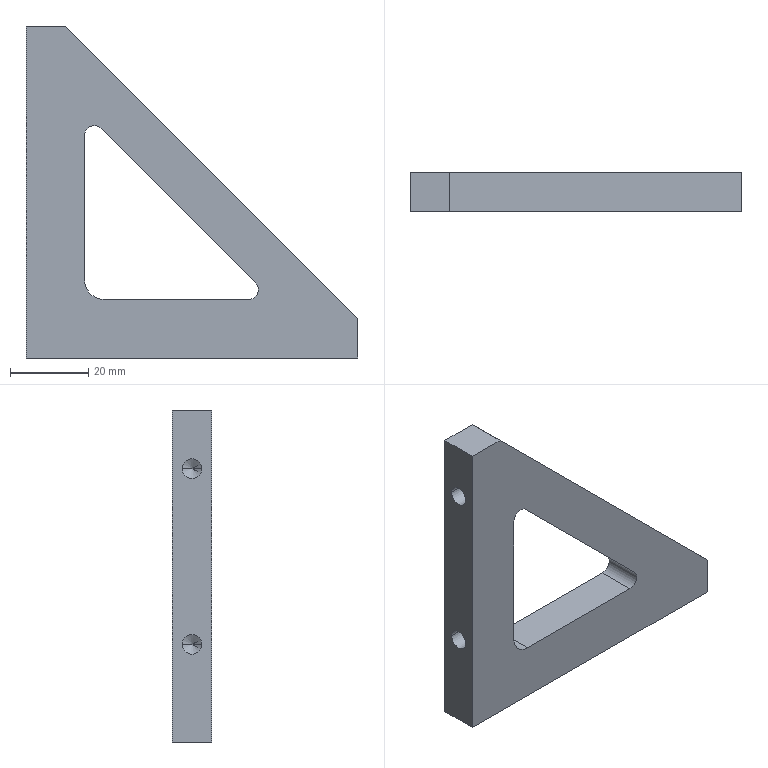Component | SolidWorks | 17081801-804-015A-1 | 1 solid | 29 faces | box 85 x 10 x 85 mm | volume 31739 mm3 | cylinder 11 | plane 10 | cone 8 | commonest cylinder face diameters 5 x10 10 x1 | material AL6061
build123d program:
from build123d import *

# Parameters (mm, degrees)
BOSS_EXTRUDE1_DEPTH   = 5
M6_TAPPED_HOLE2_D     = 5
M6_TAPPED_HOLE2_DEPTH = 13
M6_TAPPED_HOLE2_TIP   = 1.502
M6_TAPPED_HOLE1_D     = 5
M6_TAPPED_HOLE1_DEPTH = 13
M6_TAPPED_HOLE1_TIP   = 1.502
CUT_EXTRUDE1_DEPTH    = 121.623


with BuildPart() as part:
    # Sketch1 → Boss-Extrude1 (new, symmetric)
    with BuildSketch(Plane.XY):
        Polygon((0, 0), (85, 0), (85, 10), (10, 85), (0, 85), align=None)
    extrude(amount=BOSS_EXTRUDE1_DEPTH, both=True)

    # M6 Tapped Hole2
    with Locations(Plane(origin=(0, 0, 0), x_dir=(-1, 0, 0), z_dir=(0, -1, 0))):
        with Locations((-72, 0), (-27, 0)):
            Hole(M6_TAPPED_HOLE2_D / 2, depth=M6_TAPPED_HOLE2_DEPTH)
            with Locations((0, 0, -(M6_TAPPED_HOLE2_DEPTH + M6_TAPPED_HOLE2_TIP / 2))):  # 118° drill point
                Cone(0, M6_TAPPED_HOLE2_D / 2, M6_TAPPED_HOLE2_TIP, mode=Mode.SUBTRACT)

    # M6 Tapped Hole1
    with Locations(Plane(origin=(0, 0, 0), x_dir=(0, 0, -1), z_dir=(-1, 0, 0))):
        with Locations((0, -25), (0, -70)):
            Hole(M6_TAPPED_HOLE1_D / 2, depth=M6_TAPPED_HOLE1_DEPTH)
            with Locations((0, 0, -(M6_TAPPED_HOLE1_DEPTH + M6_TAPPED_HOLE1_TIP / 2))):  # 118° drill point
                Cone(0, M6_TAPPED_HOLE1_D / 2, M6_TAPPED_HOLE1_TIP, mode=Mode.SUBTRACT)

    # Sketch6 → Cut-Extrude1 (cut, through all)
    with BuildSketch(Plane(origin=(0, 0, -5), x_dir=(-1, 0, 0), z_dir=(0, 0, -1))):
        with BuildLine():
            Line((-58.762, 19.268), (-19.268, 58.762))
            ThreePointArc((-19.268, 58.762), (-16.543, 59.304), (-15, 56.994))
            Line((-15, 56.994), (-15, 20))
            ThreePointArc((-15, 20), (-16.464, 16.464), (-20, 15))
            Line((-20, 15), (-56.994, 15))
            ThreePointArc((-56.994, 15), (-59.304, 16.543), (-58.762, 19.268))
        make_face()
    extrude(amount=-CUT_EXTRUDE1_DEPTH, mode=Mode.SUBTRACT)


solid = part.part

# Placed as in the assembly
solid = solid.moved(Location((-116.5, 1974.4, 232), (90, 0, 0)))
STEP:
#1=COLOUR_RGB('',0.7922,0.8196,0.9333);
#2=FILL_AREA_STYLE_COLOUR('',#1);
#3=FILL_AREA_STYLE('',(#2));
#4=SURFACE_STYLE_FILL_AREA(#3);
#5=SURFACE_SIDE_STYLE('',(#4));
#6=SURFACE_STYLE_USAGE(.BOTH.,#5);
#7=PRESENTATION_STYLE_ASSIGNMENT((#6));
#8=CARTESIAN_POINT('',(-4.075,77.831,10.118));
#9=VERTEX_POINT('',#8);
#10=CARTESIAN_POINT('',(-4.075,77.634,10.118));
#11=VERTEX_POINT('',#10);
#12=CARTESIAN_POINT('',(-4.075,77.732,10.118));
#13=DIRECTION('',(-1.,0.,0.));
#14=DIRECTION('',(0.,-1.,0.));
#15=AXIS2_PLACEMENT_3D('',#12,#13,#14);
#16=CIRCLE('',#15,0.09843);
#17=EDGE_CURVE('',#9,#11,#16,.T.);
#18=ORIENTED_EDGE('',*,*,#17,.F.);
#19=CARTESIAN_POINT('',(-4.587,77.831,10.118));
#20=VERTEX_POINT('',#19);
#21=CARTESIAN_POINT('',(-4.587,77.831,10.118));
#22=DIRECTION('',(-1.,0.,0.));
#23=VECTOR('',#22,39.37);
#24=LINE('',#21,#23);
#25=EDGE_CURVE('',#9,#20,#24,.T.);
#26=ORIENTED_EDGE('',*,*,#25,.T.);
#27=CARTESIAN_POINT('',(-4.587,77.634,10.118));
#28=VERTEX_POINT('',#27);
#29=CARTESIAN_POINT('',(-4.587,77.732,10.118));
#30=DIRECTION('',(-1.,0.,0.));
#31=DIRECTION('',(0.,-1.,0.));
#32=AXIS2_PLACEMENT_3D('',#29,#30,#31);
#33=CIRCLE('',#32,0.09843);
#34=EDGE_CURVE('',#20,#28,#33,.T.);
#35=ORIENTED_EDGE('',*,*,#34,.T.);
#36=CARTESIAN_POINT('',(-4.587,77.634,10.118));
#37=DIRECTION('',(-1.,0.,0.));
#38=VECTOR('',#37,39.37);
#39=LINE('',#36,#38);
#40=EDGE_CURVE('',#11,#28,#39,.T.);
#41=ORIENTED_EDGE('',*,*,#40,.F.);
#42=EDGE_LOOP('',(#18,#26,#35,#41));
#43=FACE_OUTER_BOUND('',#42,.T.);
#44=CARTESIAN_POINT('',(-4.587,77.732,10.118));
#45=DIRECTION('',(-1.,0.,0.));
#46=DIRECTION('',(0.,-1.,0.));
#47=AXIS2_PLACEMENT_3D('',#44,#45,#46);
#48=CYLINDRICAL_SURFACE('',#47,0.09843);
#49=ADVANCED_FACE('',(#43),#48,.F.);
#50=CARTESIAN_POINT('',(-4.016,77.732,10.118));
#51=VERTEX_POINT('',#50);
#52=CARTESIAN_POINT('',(-4.075,77.634,10.118));
#53=DIRECTION('',(-0.515,-0.8572,-0.));
#54=VECTOR('',#53,39.37);
#55=LINE('',#52,#54);
#56=EDGE_CURVE('',#51,#11,#55,.T.);
#57=ORIENTED_EDGE('',*,*,#56,.F.);
#58=CARTESIAN_POINT('',(-4.075,77.831,10.118));
#59=DIRECTION('',(-0.515,0.8572,0.));
#60=VECTOR('',#59,39.37);
#61=LINE('',#58,#60);
#62=EDGE_CURVE('',#51,#9,#61,.T.);
#63=ORIENTED_EDGE('',*,*,#62,.T.);
#64=ORIENTED_EDGE('',*,*,#17,.T.);
#65=EDGE_LOOP('',(#57,#63,#64));
#66=FACE_OUTER_BOUND('',#65,.T.);
#67=CARTESIAN_POINT('',(-4.075,77.732,10.118));
#68=DIRECTION('',(-1.,0.,0.));
#69=DIRECTION('',(0.,-1.,0.));
#70=AXIS2_PLACEMENT_3D('',#67,#68,#69);
#71=CONICAL_SURFACE('',#70,0.09843,1.03);
#72=ADVANCED_FACE('',(#66),#71,.F.);
#73=CARTESIAN_POINT('',(-4.075,77.831,11.89));
#74=VERTEX_POINT('',#73);
#75=CARTESIAN_POINT('',(-4.075,77.634,11.89));
#76=VERTEX_POINT('',#75);
#77=CARTESIAN_POINT('',(-4.075,77.732,11.89));
#78=DIRECTION('',(-1.,0.,0.));
#79=DIRECTION('',(0.,-1.,0.));
#80=AXIS2_PLACEMENT_3D('',#77,#78,#79);
#81=CIRCLE('',#80,0.09843);
#82=EDGE_CURVE('',#74,#76,#81,.T.);
#83=ORIENTED_EDGE('',*,*,#82,.F.);
#84=CARTESIAN_POINT('',(-4.587,77.831,11.89));
#85=VERTEX_POINT('',#84);
#86=CARTESIAN_POINT('',(-4.587,77.831,11.89));
#87=DIRECTION('',(-1.,0.,0.));
#88=VECTOR('',#87,39.37);
#89=LINE('',#86,#88);
#90=EDGE_CURVE('',#74,#85,#89,.T.);
#91=ORIENTED_EDGE('',*,*,#90,.T.);
#92=CARTESIAN_POINT('',(-4.587,77.634,11.89));
#93=VERTEX_POINT('',#92);
#94=CARTESIAN_POINT('',(-4.587,77.732,11.89));
#95=DIRECTION('',(-1.,0.,0.));
#96=DIRECTION('',(0.,-1.,0.));
#97=AXIS2_PLACEMENT_3D('',#94,#95,#96);
#98=CIRCLE('',#97,0.09843);
#99=EDGE_CURVE('',#85,#93,#98,.T.);
#100=ORIENTED_EDGE('',*,*,#99,.T.);
#101=CARTESIAN_POINT('',(-4.587,77.634,11.89));
#102=DIRECTION('',(-1.,0.,0.));
#103=VECTOR('',#102,39.37);
#104=LINE('',#101,#103);
#105=EDGE_CURVE('',#76,#93,#104,.T.);
#106=ORIENTED_EDGE('',*,*,#105,.F.);
#107=EDGE_LOOP('',(#83,#91,#100,#106));
#108=FACE_OUTER_BOUND('',#107,.T.);
#109=CARTESIAN_POINT('',(-4.587,77.732,11.89));
#110=DIRECTION('',(-1.,0.,0.));
#111=DIRECTION('',(0.,-1.,0.));
#112=AXIS2_PLACEMENT_3D('',#109,#110,#111);
#113=CYLINDRICAL_SURFACE('',#112,0.09843);
#114=ADVANCED_FACE('',(#108),#113,.F.);
#115=CARTESIAN_POINT('',(-4.016,77.732,11.89));
#116=VERTEX_POINT('',#115);
#117=CARTESIAN_POINT('',(-4.075,77.634,11.89));
#118=DIRECTION('',(-0.515,-0.8572,-0.));
#119=VECTOR('',#118,39.37);
#120=LINE('',#117,#119);
#121=EDGE_CURVE('',#116,#76,#120,.T.);
#122=ORIENTED_EDGE('',*,*,#121,.F.);
#123=CARTESIAN_POINT('',(-4.075,77.831,11.89));
#124=DIRECTION('',(-0.515,0.8572,0.));
#125=VECTOR('',#124,39.37);
#126=LINE('',#123,#125);
#127=EDGE_CURVE('',#116,#74,#126,.T.);
#128=ORIENTED_EDGE('',*,*,#127,.T.);
#129=ORIENTED_EDGE('',*,*,#82,.T.);
#130=EDGE_LOOP('',(#122,#128,#129));
#131=FACE_OUTER_BOUND('',#130,.T.);
#132=CARTESIAN_POINT('',(-4.075,77.732,11.89));
#133=DIRECTION('',(-1.,0.,0.));
#134=DIRECTION('',(0.,-1.,0.));
#135=AXIS2_PLACEMENT_3D('',#132,#133,#134);
#136=CONICAL_SURFACE('',#135,0.09843,1.03);
#137=ADVANCED_FACE('',(#131),#136,.F.);
#138=CARTESIAN_POINT('',(-1.752,77.634,9.646));
#139=VERTEX_POINT('',#138);
#140=CARTESIAN_POINT('',(-1.752,77.831,9.646));
#141=VERTEX_POINT('',#140);
#142=CARTESIAN_POINT('',(-1.752,77.732,9.646));
#143=DIRECTION('',(-0.,0.,-1.));
#144=DIRECTION('',(0.,1.,0.));
#145=AXIS2_PLACEMENT_3D('',#142,#143,#144);
#146=CIRCLE('',#145,0.09843);
#147=EDGE_CURVE('',#139,#141,#146,.T.);
#148=ORIENTED_EDGE('',*,*,#147,.F.);
#149=CARTESIAN_POINT('',(-1.752,77.634,9.134));
#150=VERTEX_POINT('',#149);
#151=CARTESIAN_POINT('',(-1.752,77.634,9.134));
#152=DIRECTION('',(-0.,0.,-1.));
#153=VECTOR('',#152,39.37);
#154=LINE('',#151,#153);
#155=EDGE_CURVE('',#139,#150,#154,.T.);
#156=ORIENTED_EDGE('',*,*,#155,.T.);
#157=CARTESIAN_POINT('',(-1.752,77.831,9.134));
#158=VERTEX_POINT('',#157);
#159=CARTESIAN_POINT('',(-1.752,77.732,9.134));
#160=DIRECTION('',(-0.,0.,-1.));
#161=DIRECTION('',(0.,1.,0.));
#162=AXIS2_PLACEMENT_3D('',#159,#160,#161);
#163=CIRCLE('',#162,0.09843);
#164=EDGE_CURVE('',#150,#158,#163,.T.);
#165=ORIENTED_EDGE('',*,*,#164,.T.);
#166=CARTESIAN_POINT('',(-1.752,77.831,9.134));
#167=DIRECTION('',(-0.,0.,-1.));
#168=VECTOR('',#167,39.37);
#169=LINE('',#166,#168);
#170=EDGE_CURVE('',#141,#158,#169,.T.);
#171=ORIENTED_EDGE('',*,*,#170,.F.);
#172=EDGE_LOOP('',(#148,#156,#165,#171));
#173=FACE_OUTER_BOUND('',#172,.T.);
#174=CARTESIAN_POINT('',(-1.752,77.732,9.134));
#175=DIRECTION('',(-0.,0.,-1.));
#176=DIRECTION('',(0.,1.,0.));
#177=AXIS2_PLACEMENT_3D('',#174,#175,#176);
#178=CYLINDRICAL_SURFACE('',#177,0.09843);
#179=ADVANCED_FACE('',(#173),#178,.F.);
#180=CARTESIAN_POINT('',(-1.752,77.732,9.705));
#181=VERTEX_POINT('',#180);
#182=CARTESIAN_POINT('',(-1.752,77.831,9.646));
#183=DIRECTION('',(0.,0.8572,-0.515));
#184=VECTOR('',#183,39.37);
#185=LINE('',#182,#184);
#186=EDGE_CURVE('',#181,#141,#185,.T.);
#187=ORIENTED_EDGE('',*,*,#186,.F.);
#188=CARTESIAN_POINT('',(-1.752,77.634,9.646));
#189=DIRECTION('',(-0.,-0.8572,-0.515));
#190=VECTOR('',#189,39.37);
#191=LINE('',#188,#190);
#192=EDGE_CURVE('',#181,#139,#191,.T.);
#193=ORIENTED_EDGE('',*,*,#192,.T.);
#194=ORIENTED_EDGE('',*,*,#147,.T.);
#195=EDGE_LOOP('',(#187,#193,#194));
#196=FACE_OUTER_BOUND('',#195,.T.);
#197=CARTESIAN_POINT('',(-1.752,77.732,9.646));
#198=DIRECTION('',(-0.,0.,-1.));
#199=DIRECTION('',(0.,1.,0.));
#200=AXIS2_PLACEMENT_3D('',#197,#198,#199);
#201=CONICAL_SURFACE('',#200,0.09843,1.03);
#202=ADVANCED_FACE('',(#196),#201,.F.);
#203=CARTESIAN_POINT('',(-3.524,77.634,9.646));
#204=VERTEX_POINT('',#203);
#205=CARTESIAN_POINT('',(-3.524,77.831,9.646));
#206=VERTEX_POINT('',#205);
#207=CARTESIAN_POINT('',(-3.524,77.732,9.646));
#208=DIRECTION('',(-0.,0.,-1.));
#209=DIRECTION('',(0.,1.,0.));
#210=AXIS2_PLACEMENT_3D('',#207,#208,#209);
#211=CIRCLE('',#210,0.09843);
#212=EDGE_CURVE('',#204,#206,#211,.T.);
#213=ORIENTED_EDGE('',*,*,#212,.F.);
#214=CARTESIAN_POINT('',(-3.524,77.634,9.134));
#215=VERTEX_POINT('',#214);
#216=CARTESIAN_POINT('',(-3.524,77.634,9.134));
#217=DIRECTION('',(-0.,0.,-1.));
#218=VECTOR('',#217,39.37);
#219=LINE('',#216,#218);
#220=EDGE_CURVE('',#204,#215,#219,.T.);
#221=ORIENTED_EDGE('',*,*,#220,.T.);
#222=CARTESIAN_POINT('',(-3.524,77.831,9.134));
#223=VERTEX_POINT('',#222);
#224=CARTESIAN_POINT('',(-3.524,77.732,9.134));
#225=DIRECTION('',(-0.,0.,-1.));
#226=DIRECTION('',(0.,1.,0.));
#227=AXIS2_PLACEMENT_3D('',#224,#225,#226);
#228=CIRCLE('',#227,0.09843);
#229=EDGE_CURVE('',#215,#223,#228,.T.);
#230=ORIENTED_EDGE('',*,*,#229,.T.);
#231=CARTESIAN_POINT('',(-3.524,77.831,9.134));
#232=DIRECTION('',(-0.,0.,-1.));
#233=VECTOR('',#232,39.37);
#234=LINE('',#231,#233);
#235=EDGE_CURVE('',#206,#223,#234,.T.);
#236=ORIENTED_EDGE('',*,*,#235,.F.);
#237=EDGE_LOOP('',(#213,#221,#230,#236));
#238=FACE_OUTER_BOUND('',#237,.T.);
#239=CARTESIAN_POINT('',(-3.524,77.732,9.134));
#240=DIRECTION('',(-0.,0.,-1.));
#241=DIRECTION('',(0.,1.,0.));
#242=AXIS2_PLACEMENT_3D('',#239,#240,#241);
#243=CYLINDRICAL_SURFACE('',#242,0.09843);
#244=ADVANCED_FACE('',(#238),#243,.F.);
#245=CARTESIAN_POINT('',(-3.524,77.732,9.705));
#246=VERTEX_POINT('',#245);
#247=CARTESIAN_POINT('',(-3.524,77.831,9.646));
#248=DIRECTION('',(0.,0.8572,-0.515));
#249=VECTOR('',#248,39.37);
#250=LINE('',#247,#249);
#251=EDGE_CURVE('',#246,#206,#250,.T.);
#252=ORIENTED_EDGE('',*,*,#251,.F.);
#253=CARTESIAN_POINT('',(-3.524,77.634,9.646));
#254=DIRECTION('',(-0.,-0.8572,-0.515));
#255=VECTOR('',#254,39.37);
#256=LINE('',#253,#255);
#257=EDGE_CURVE('',#246,#204,#256,.T.);
#258=ORIENTED_EDGE('',*,*,#257,.T.);
#259=ORIENTED_EDGE('',*,*,#212,.T.);
#260=EDGE_LOOP('',(#252,#258,#259));
#261=FACE_OUTER_BOUND('',#260,.T.);
#262=CARTESIAN_POINT('',(-3.524,77.732,9.646));
#263=DIRECTION('',(-0.,0.,-1.));
#264=DIRECTION('',(0.,1.,0.));
#265=AXIS2_PLACEMENT_3D('',#262,#263,#264);
#266=CONICAL_SURFACE('',#265,0.09843,1.03);
#267=ADVANCED_FACE('',(#261),#266,.F.);
#268=CARTESIAN_POINT('',(-4.587,77.732,10.118));
#269=DIRECTION('',(-1.,0.,0.));
#270=DIRECTION('',(0.,-1.,0.));
#271=AXIS2_PLACEMENT_3D('',#268,#269,#270);
#272=CIRCLE('',#271,0.09843);
#273=EDGE_CURVE('',#28,#20,#272,.T.);
#274=ORIENTED_EDGE('',*,*,#273,.F.);
#275=ORIENTED_EDGE('',*,*,#34,.F.);
#276=EDGE_LOOP('',(#274,#275));
#277=FACE_BOUND('',#276,.T.);
#278=CARTESIAN_POINT('',(-4.587,77.732,11.89));
#279=DIRECTION('',(-1.,0.,0.));
#280=DIRECTION('',(0.,-1.,0.));
#281=AXIS2_PLACEMENT_3D('',#278,#279,#280);
#282=CIRCLE('',#281,0.09843);
#283=EDGE_CURVE('',#93,#85,#282,.T.);
#284=ORIENTED_EDGE('',*,*,#283,.F.);
#285=ORIENTED_EDGE('',*,*,#99,.F.);
#286=EDGE_LOOP('',(#284,#285));
#287=FACE_BOUND('',#286,.T.);
#288=CARTESIAN_POINT('',(-4.587,77.929,12.48));
#289=VERTEX_POINT('',#288);
#290=CARTESIAN_POINT('',(-4.587,77.929,9.134));
#291=VERTEX_POINT('',#290);
#292=CARTESIAN_POINT('',(-4.587,77.929,12.48));
#293=DIRECTION('',(-0.,0.,-1.));
#294=VECTOR('',#293,39.37);
#295=LINE('',#292,#294);
#296=EDGE_CURVE('',#289,#291,#295,.T.);
#297=ORIENTED_EDGE('',*,*,#296,.T.);
#298=CARTESIAN_POINT('',(-4.587,77.535,9.134));
#299=VERTEX_POINT('',#298);
#300=CARTESIAN_POINT('',(-4.587,77.535,9.134));
#301=DIRECTION('',(0.,1.,0.));
#302=VECTOR('',#301,39.37);
#303=LINE('',#300,#302);
#304=EDGE_CURVE('',#299,#291,#303,.T.);
#305=ORIENTED_EDGE('',*,*,#304,.F.);
#306=CARTESIAN_POINT('',(-4.587,77.535,12.48));
#307=VERTEX_POINT('',#306);
#308=CARTESIAN_POINT('',(-4.587,77.535,12.48));
#309=DIRECTION('',(-0.,0.,-1.));
#310=VECTOR('',#309,39.37);
#311=LINE('',#308,#310);
#312=EDGE_CURVE('',#307,#299,#311,.T.);
#313=ORIENTED_EDGE('',*,*,#312,.F.);
#314=CARTESIAN_POINT('',(-4.587,77.535,12.48));
#315=DIRECTION('',(0.,1.,0.));
#316=VECTOR('',#315,39.37);
#317=LINE('',#314,#316);
#318=EDGE_CURVE('',#307,#289,#317,.T.);
#319=ORIENTED_EDGE('',*,*,#318,.T.);
#320=EDGE_LOOP('',(#297,#305,#313,#319));
#321=FACE_OUTER_BOUND('',#320,.T.);
#322=CARTESIAN_POINT('',(-4.587,77.535,12.48));
#323=DIRECTION('',(1.,-0.,-0.));
#324=DIRECTION('',(0.,-0.,1.));
#325=AXIS2_PLACEMENT_3D('',#322,#323,#324);
#326=PLANE('',#325);
#327=ADVANCED_FACE('',(#277,#287,#321),#326,.F.);
#328=CARTESIAN_POINT('',(-1.752,77.732,9.134));
#329=DIRECTION('',(-0.,0.,-1.));
#330=DIRECTION('',(0.,1.,0.));
#331=AXIS2_PLACEMENT_3D('',#328,#329,#330);
#332=CIRCLE('',#331,0.09843);
#333=EDGE_CURVE('',#158,#150,#332,.T.);
#334=ORIENTED_EDGE('',*,*,#333,.F.);
#335=ORIENTED_EDGE('',*,*,#164,.F.);
#336=EDGE_LOOP('',(#334,#335));
#337=FACE_BOUND('',#336,.T.);
#338=CARTESIAN_POINT('',(-3.524,77.732,9.134));
#339=DIRECTION('',(-0.,0.,-1.));
#340=DIRECTION('',(0.,1.,0.));
#341=AXIS2_PLACEMENT_3D('',#338,#339,#340);
#342=CIRCLE('',#341,0.09843);
#343=EDGE_CURVE('',#223,#215,#342,.T.);
#344=ORIENTED_EDGE('',*,*,#343,.F.);
#345=ORIENTED_EDGE('',*,*,#229,.F.);
#346=EDGE_LOOP('',(#344,#345));
#347=FACE_BOUND('',#346,.T.);
#348=CARTESIAN_POINT('',(-1.24,77.929,9.134));
#349=VERTEX_POINT('',#348);
#350=CARTESIAN_POINT('',(-4.587,77.929,9.134));
#351=DIRECTION('',(1.,-0.,-0.));
#352=VECTOR('',#351,39.37);
#353=LINE('',#350,#352);
#354=EDGE_CURVE('',#291,#349,#353,.T.);
#355=ORIENTED_EDGE('',*,*,#354,.T.);
#356=CARTESIAN_POINT('',(-1.24,77.535,9.134));
#357=VERTEX_POINT('',#356);
#358=CARTESIAN_POINT('',(-1.24,77.535,9.134));
#359=DIRECTION('',(0.,1.,0.));
#360=VECTOR('',#359,39.37);
#361=LINE('',#358,#360);
#362=EDGE_CURVE('',#357,#349,#361,.T.);
#363=ORIENTED_EDGE('',*,*,#362,.F.);
#364=CARTESIAN_POINT('',(-4.587,77.535,9.134));
#365=DIRECTION('',(1.,-0.,-0.));
#366=VECTOR('',#365,39.37);
#367=LINE('',#364,#366);
#368=EDGE_CURVE('',#299,#357,#367,.T.);
#369=ORIENTED_EDGE('',*,*,#368,.F.);
#370=ORIENTED_EDGE('',*,*,#304,.T.);
#371=EDGE_LOOP('',(#355,#363,#369,#370));
#372=FACE_OUTER_BOUND('',#371,.T.);
#373=CARTESIAN_POINT('',(-4.587,77.535,9.134));
#374=DIRECTION('',(0.,-0.,1.));
#375=DIRECTION('',(-0.,-1.,-0.));
#376=AXIS2_PLACEMENT_3D('',#373,#374,#375);
#377=PLANE('',#376);
#378=ADVANCED_FACE('',(#337,#347,#372),#377,.F.);
#379=CARTESIAN_POINT('',(-1.24,77.929,9.528));
#380=VERTEX_POINT('',#379);
#381=CARTESIAN_POINT('',(-1.24,77.929,9.134));
#382=DIRECTION('',(0.,-0.,1.));
#383=VECTOR('',#382,39.37);
#384=LINE('',#381,#383);
#385=EDGE_CURVE('',#349,#380,#384,.T.);
#386=ORIENTED_EDGE('',*,*,#385,.T.);
#387=CARTESIAN_POINT('',(-1.24,77.535,9.528));
#388=VERTEX_POINT('',#387);
#389=CARTESIAN_POINT('',(-1.24,77.535,9.528));
#390=DIRECTION('',(0.,1.,0.));
#391=VECTOR('',#390,39.37);
#392=LINE('',#389,#391);
#393=EDGE_CURVE('',#388,#380,#392,.T.);
#394=ORIENTED_EDGE('',*,*,#393,.F.);
#395=CARTESIAN_POINT('',(-1.24,77.535,9.134));
#396=DIRECTION('',(0.,-0.,1.));
#397=VECTOR('',#396,39.37);
#398=LINE('',#395,#397);
#399=EDGE_CURVE('',#357,#388,#398,.T.);
#400=ORIENTED_EDGE('',*,*,#399,.F.);
#401=ORIENTED_EDGE('',*,*,#362,.T.);
#402=EDGE_LOOP('',(#386,#394,#400,#401));
#403=FACE_OUTER_BOUND('',#402,.T.);
#404=CARTESIAN_POINT('',(-1.24,77.535,9.134));
#405=DIRECTION('',(-1.,0.,0.));
#406=DIRECTION('',(-0.,-1.,-0.));
#407=AXIS2_PLACEMENT_3D('',#404,#405,#406);
#408=PLANE('',#407);
#409=ADVANCED_FACE('',(#403),#408,.F.);
#410=CARTESIAN_POINT('',(-4.193,77.929,12.48));
#411=VERTEX_POINT('',#410);
#412=CARTESIAN_POINT('',(-1.24,77.929,9.528));
#413=DIRECTION('',(-0.7071,0.,0.7071));
#414=VECTOR('',#413,39.37);
#415=LINE('',#412,#414);
#416=EDGE_CURVE('',#380,#411,#415,.T.);
#417=ORIENTED_EDGE('',*,*,#416,.T.);
#418=CARTESIAN_POINT('',(-4.193,77.535,12.48));
#419=VERTEX_POINT('',#418);
#420=CARTESIAN_POINT('',(-4.193,77.535,12.48));
#421=DIRECTION('',(0.,1.,0.));
#422=VECTOR('',#421,39.37);
#423=LINE('',#420,#422);
#424=EDGE_CURVE('',#419,#411,#423,.T.);
#425=ORIENTED_EDGE('',*,*,#424,.F.);
#426=CARTESIAN_POINT('',(-1.24,77.535,9.528));
#427=DIRECTION('',(-0.7071,0.,0.7071));
#428=VECTOR('',#427,39.37);
#429=LINE('',#426,#428);
#430=EDGE_CURVE('',#388,#419,#429,.T.);
#431=ORIENTED_EDGE('',*,*,#430,.F.);
#432=ORIENTED_EDGE('',*,*,#393,.T.);
#433=EDGE_LOOP('',(#417,#425,#431,#432));
#434=FACE_OUTER_BOUND('',#433,.T.);
#435=CARTESIAN_POINT('',(-1.24,77.535,9.528));
#436=DIRECTION('',(-0.7071,0.,-0.7071));
#437=DIRECTION('',(0.7071,-0.,-0.7071));
#438=AXIS2_PLACEMENT_3D('',#435,#436,#437);
#439=PLANE('',#438);
#440=ADVANCED_FACE('',(#434),#439,.F.);
#441=CARTESIAN_POINT('',(-4.193,77.929,12.48));
#442=DIRECTION('',(-1.,0.,0.));
#443=VECTOR('',#442,39.37);
#444=LINE('',#441,#443);
#445=EDGE_CURVE('',#411,#289,#444,.T.);
#446=ORIENTED_EDGE('',*,*,#445,.T.);
#447=ORIENTED_EDGE('',*,*,#318,.F.);
#448=CARTESIAN_POINT('',(-4.193,77.535,12.48));
#449=DIRECTION('',(-1.,0.,0.));
#450=VECTOR('',#449,39.37);
#451=LINE('',#448,#450);
#452=EDGE_CURVE('',#419,#307,#451,.T.);
#453=ORIENTED_EDGE('',*,*,#452,.F.);
#454=ORIENTED_EDGE('',*,*,#424,.T.);
#455=EDGE_LOOP('',(#446,#447,#453,#454));
#456=FACE_OUTER_BOUND('',#455,.T.);
#457=CARTESIAN_POINT('',(-4.193,77.535,12.48));
#458=DIRECTION('',(-0.,0.,-1.));
#459=DIRECTION('',(0.,1.,0.));
#460=AXIS2_PLACEMENT_3D('',#457,#458,#459);
#461=PLANE('',#460);
#462=ADVANCED_FACE('',(#456),#461,.F.);
#463=CARTESIAN_POINT('',(-3.799,77.535,9.724));
#464=VERTEX_POINT('',#463);
#465=CARTESIAN_POINT('',(-3.996,77.535,9.921));
#466=VERTEX_POINT('',#465);
#467=CARTESIAN_POINT('',(-3.799,77.535,9.921));
#468=DIRECTION('',(0.,1.,0.));
#469=DIRECTION('',(1.,0.,0.));
#470=AXIS2_PLACEMENT_3D('',#467,#468,#469);
#471=CIRCLE('',#470,0.1969);
#472=EDGE_CURVE('',#464,#466,#471,.T.);
#473=ORIENTED_EDGE('',*,*,#472,.T.);
#474=CARTESIAN_POINT('',(-3.996,77.535,11.378));
#475=VERTEX_POINT('',#474);
#476=CARTESIAN_POINT('',(-3.996,77.535,11.378));
#477=DIRECTION('',(0.,-0.,1.));
#478=VECTOR('',#477,39.37);
#479=LINE('',#476,#478);
#480=EDGE_CURVE('',#466,#475,#479,.T.);
#481=ORIENTED_EDGE('',*,*,#480,.T.);
#482=CARTESIAN_POINT('',(-3.828,77.535,11.447));
#483=VERTEX_POINT('',#482);
#484=CARTESIAN_POINT('',(-3.898,77.535,11.378));
#485=DIRECTION('',(0.,1.,0.));
#486=DIRECTION('',(-1.,0.,0.));
#487=AXIS2_PLACEMENT_3D('',#484,#485,#486);
#488=CIRCLE('',#487,0.09843);
#489=EDGE_CURVE('',#475,#483,#488,.T.);
#490=ORIENTED_EDGE('',*,*,#489,.T.);
#491=CARTESIAN_POINT('',(-2.273,77.535,9.892));
#492=VERTEX_POINT('',#491);
#493=CARTESIAN_POINT('',(-2.273,77.535,9.892));
#494=DIRECTION('',(0.7071,-0.,-0.7071));
#495=VECTOR('',#494,39.37);
#496=LINE('',#493,#495);
#497=EDGE_CURVE('',#483,#492,#496,.T.);
#498=ORIENTED_EDGE('',*,*,#497,.T.);
#499=CARTESIAN_POINT('',(-2.343,77.535,9.724));
#500=VERTEX_POINT('',#499);
#501=CARTESIAN_POINT('',(-2.343,77.535,9.823));
#502=DIRECTION('',(0.,1.,0.));
#503=DIRECTION('',(-1.,0.,0.));
#504=AXIS2_PLACEMENT_3D('',#501,#502,#503);
#505=CIRCLE('',#504,0.09843);
#506=EDGE_CURVE('',#492,#500,#505,.T.);
#507=ORIENTED_EDGE('',*,*,#506,.T.);
#508=CARTESIAN_POINT('',(-3.799,77.535,9.724));
#509=DIRECTION('',(-1.,0.,0.));
#510=VECTOR('',#509,39.37);
#511=LINE('',#508,#510);
#512=EDGE_CURVE('',#500,#464,#511,.T.);
#513=ORIENTED_EDGE('',*,*,#512,.T.);
#514=EDGE_LOOP('',(#473,#481,#490,#498,#507,#513));
#515=FACE_BOUND('',#514,.T.);
#516=ORIENTED_EDGE('',*,*,#312,.T.);
#517=ORIENTED_EDGE('',*,*,#368,.T.);
#518=ORIENTED_EDGE('',*,*,#399,.T.);
#519=ORIENTED_EDGE('',*,*,#430,.T.);
#520=ORIENTED_EDGE('',*,*,#452,.T.);
#521=EDGE_LOOP('',(#516,#517,#518,#519,#520));
#522=FACE_OUTER_BOUND('',#521,.T.);
#523=CARTESIAN_POINT('',(-4.587,77.535,9.134));
#524=DIRECTION('',(-0.,-1.,-0.));
#525=DIRECTION('',(1.,-0.,-0.));
#526=AXIS2_PLACEMENT_3D('',#523,#524,#525);
#527=PLANE('',#526);
#528=ADVANCED_FACE('',(#515,#522),#527,.T.);
#529=CARTESIAN_POINT('',(-3.996,77.929,9.921));
#530=VERTEX_POINT('',#529);
#531=CARTESIAN_POINT('',(-3.996,77.929,11.378));
#532=VERTEX_POINT('',#531);
#533=CARTESIAN_POINT('',(-3.996,77.929,11.378));
#534=DIRECTION('',(0.,-0.,1.));
#535=VECTOR('',#534,39.37);
#536=LINE('',#533,#535);
#537=EDGE_CURVE('',#530,#532,#536,.T.);
#538=ORIENTED_EDGE('',*,*,#537,.F.);
#539=CARTESIAN_POINT('',(-3.799,77.929,9.724));
#540=VERTEX_POINT('',#539);
#541=CARTESIAN_POINT('',(-3.799,77.929,9.921));
#542=DIRECTION('',(0.,1.,0.));
#543=DIRECTION('',(1.,0.,0.));
#544=AXIS2_PLACEMENT_3D('',#541,#542,#543);
#545=CIRCLE('',#544,0.1969);
#546=EDGE_CURVE('',#540,#530,#545,.T.);
#547=ORIENTED_EDGE('',*,*,#546,.F.);
#548=CARTESIAN_POINT('',(-2.343,77.929,9.724));
#549=VERTEX_POINT('',#548);
#550=CARTESIAN_POINT('',(-3.799,77.929,9.724));
#551=DIRECTION('',(-1.,0.,0.));
#552=VECTOR('',#551,39.37);
#553=LINE('',#550,#552);
#554=EDGE_CURVE('',#549,#540,#553,.T.);
#555=ORIENTED_EDGE('',*,*,#554,.F.);
#556=CARTESIAN_POINT('',(-2.273,77.929,9.892));
#557=VERTEX_POINT('',#556);
#558=CARTESIAN_POINT('',(-2.343,77.929,9.823));
#559=DIRECTION('',(0.,1.,0.));
#560=DIRECTION('',(-1.,0.,0.));
#561=AXIS2_PLACEMENT_3D('',#558,#559,#560);
#562=CIRCLE('',#561,0.09843);
#563=EDGE_CURVE('',#557,#549,#562,.T.);
#564=ORIENTED_EDGE('',*,*,#563,.F.);
#565=CARTESIAN_POINT('',(-3.828,77.929,11.447));
#566=VERTEX_POINT('',#565);
#567=CARTESIAN_POINT('',(-2.273,77.929,9.892));
#568=DIRECTION('',(0.7071,-0.,-0.7071));
#569=VECTOR('',#568,39.37);
#570=LINE('',#567,#569);
#571=EDGE_CURVE('',#566,#557,#570,.T.);
#572=ORIENTED_EDGE('',*,*,#571,.F.);
#573=CARTESIAN_POINT('',(-3.898,77.929,11.378));
#574=DIRECTION('',(0.,1.,0.));
#575=DIRECTION('',(-1.,0.,0.));
#576=AXIS2_PLACEMENT_3D('',#573,#574,#575);
#577=CIRCLE('',#576,0.09843);
#578=EDGE_CURVE('',#532,#566,#577,.T.);
#579=ORIENTED_EDGE('',*,*,#578,.F.);
#580=EDGE_LOOP('',(#538,#547,#555,#564,#572,#579));
#581=FACE_BOUND('',#580,.T.);
#582=ORIENTED_EDGE('',*,*,#296,.F.);
#583=ORIENTED_EDGE('',*,*,#445,.F.);
#584=ORIENTED_EDGE('',*,*,#416,.F.);
#585=ORIENTED_EDGE('',*,*,#385,.F.);
#586=ORIENTED_EDGE('',*,*,#354,.F.);
#587=EDGE_LOOP('',(#582,#583,#584,#585,#586));
#588=FACE_OUTER_BOUND('',#587,.T.);
#589=CARTESIAN_POINT('',(-4.587,77.929,9.134));
#590=DIRECTION('',(-0.,-1.,-0.));
#591=DIRECTION('',(1.,-0.,-0.));
#592=AXIS2_PLACEMENT_3D('',#589,#590,#591);
#593=PLANE('',#592);
#594=ADVANCED_FACE('',(#581,#588),#593,.F.);
#595=ORIENTED_EDGE('',*,*,#257,.F.);
#596=ORIENTED_EDGE('',*,*,#251,.T.);
#597=CARTESIAN_POINT('',(-3.524,77.732,9.646));
#598=DIRECTION('',(-0.,0.,-1.));
#599=DIRECTION('',(0.,1.,0.));
#600=AXIS2_PLACEMENT_3D('',#597,#598,#599);
#601=CIRCLE('',#600,0.09843);
#602=EDGE_CURVE('',#206,#204,#601,.T.);
#603=ORIENTED_EDGE('',*,*,#602,.T.);
#604=EDGE_LOOP('',(#595,#596,#603));
#605=FACE_OUTER_BOUND('',#604,.T.);
#606=CARTESIAN_POINT('',(-3.524,77.732,9.646));
#607=DIRECTION('',(-0.,0.,-1.));
#608=DIRECTION('',(0.,1.,0.));
#609=AXIS2_PLACEMENT_3D('',#606,#607,#608);
#610=CONICAL_SURFACE('',#609,0.09843,1.03);
#611=ADVANCED_FACE('',(#605),#610,.F.);
#612=ORIENTED_EDGE('',*,*,#220,.F.);
#613=ORIENTED_EDGE('',*,*,#602,.F.);
#614=ORIENTED_EDGE('',*,*,#235,.T.);
#615=ORIENTED_EDGE('',*,*,#343,.T.);
#616=EDGE_LOOP('',(#612,#613,#614,#615));
#617=FACE_OUTER_BOUND('',#616,.T.);
#618=CARTESIAN_POINT('',(-3.524,77.732,9.134));
#619=DIRECTION('',(-0.,0.,-1.));
#620=DIRECTION('',(0.,1.,0.));
#621=AXIS2_PLACEMENT_3D('',#618,#619,#620);
#622=CYLINDRICAL_SURFACE('',#621,0.09843);
#623=ADVANCED_FACE('',(#617),#622,.F.);
#624=ORIENTED_EDGE('',*,*,#192,.F.);
#625=ORIENTED_EDGE('',*,*,#186,.T.);
#626=CARTESIAN_POINT('',(-1.752,77.732,9.646));
#627=DIRECTION('',(-0.,0.,-1.));
#628=DIRECTION('',(0.,1.,0.));
#629=AXIS2_PLACEMENT_3D('',#626,#627,#628);
#630=CIRCLE('',#629,0.09843);
#631=EDGE_CURVE('',#141,#139,#630,.T.);
#632=ORIENTED_EDGE('',*,*,#631,.T.);
#633=EDGE_LOOP('',(#624,#625,#632));
#634=FACE_OUTER_BOUND('',#633,.T.);
#635=CARTESIAN_POINT('',(-1.752,77.732,9.646));
#636=DIRECTION('',(-0.,0.,-1.));
#637=DIRECTION('',(0.,1.,0.));
#638=AXIS2_PLACEMENT_3D('',#635,#636,#637);
#639=CONICAL_SURFACE('',#638,0.09843,1.03);
#640=ADVANCED_FACE('',(#634),#639,.F.);
#641=ORIENTED_EDGE('',*,*,#155,.F.);
#642=ORIENTED_EDGE('',*,*,#631,.F.);
#643=ORIENTED_EDGE('',*,*,#170,.T.);
#644=ORIENTED_EDGE('',*,*,#333,.T.);
#645=EDGE_LOOP('',(#641,#642,#643,#644));
#646=FACE_OUTER_BOUND('',#645,.T.);
#647=CARTESIAN_POINT('',(-1.752,77.732,9.134));
#648=DIRECTION('',(-0.,0.,-1.));
#649=DIRECTION('',(0.,1.,0.));
#650=AXIS2_PLACEMENT_3D('',#647,#648,#649);
#651=CYLINDRICAL_SURFACE('',#650,0.09843);
#652=ADVANCED_FACE('',(#646),#651,.F.);
#653=ORIENTED_EDGE('',*,*,#127,.F.);
#654=ORIENTED_EDGE('',*,*,#121,.T.);
#655=CARTESIAN_POINT('',(-4.075,77.732,11.89));
#656=DIRECTION('',(-1.,0.,0.));
#657=DIRECTION('',(0.,-1.,0.));
#658=AXIS2_PLACEMENT_3D('',#655,#656,#657);
#659=CIRCLE('',#658,0.09843);
#660=EDGE_CURVE('',#76,#74,#659,.T.);
#661=ORIENTED_EDGE('',*,*,#660,.T.);
#662=EDGE_LOOP('',(#653,#654,#661));
#663=FACE_OUTER_BOUND('',#662,.T.);
#664=CARTESIAN_POINT('',(-4.075,77.732,11.89));
#665=DIRECTION('',(-1.,0.,0.));
#666=DIRECTION('',(0.,-1.,0.));
#667=AXIS2_PLACEMENT_3D('',#664,#665,#666);
#668=CONICAL_SURFACE('',#667,0.09843,1.03);
#669=ADVANCED_FACE('',(#663),#668,.F.);
#670=ORIENTED_EDGE('',*,*,#90,.F.);
#671=ORIENTED_EDGE('',*,*,#660,.F.);
#672=ORIENTED_EDGE('',*,*,#105,.T.);
#673=ORIENTED_EDGE('',*,*,#283,.T.);
#674=EDGE_LOOP('',(#670,#671,#672,#673));
#675=FACE_OUTER_BOUND('',#674,.T.);
#676=CARTESIAN_POINT('',(-4.587,77.732,11.89));
#677=DIRECTION('',(-1.,0.,0.));
#678=DIRECTION('',(0.,-1.,0.));
#679=AXIS2_PLACEMENT_3D('',#676,#677,#678);
#680=CYLINDRICAL_SURFACE('',#679,0.09843);
#681=ADVANCED_FACE('',(#675),#680,.F.);
#682=ORIENTED_EDGE('',*,*,#62,.F.);
#683=ORIENTED_EDGE('',*,*,#56,.T.);
#684=CARTESIAN_POINT('',(-4.075,77.732,10.118));
#685=DIRECTION('',(-1.,0.,0.));
#686=DIRECTION('',(0.,-1.,0.));
#687=AXIS2_PLACEMENT_3D('',#684,#685,#686);
#688=CIRCLE('',#687,0.09843);
#689=EDGE_CURVE('',#11,#9,#688,.T.);
#690=ORIENTED_EDGE('',*,*,#689,.T.);
#691=EDGE_LOOP('',(#682,#683,#690));
#692=FACE_OUTER_BOUND('',#691,.T.);
#693=CARTESIAN_POINT('',(-4.075,77.732,10.118));
#694=DIRECTION('',(-1.,0.,0.));
#695=DIRECTION('',(0.,-1.,0.));
#696=AXIS2_PLACEMENT_3D('',#693,#694,#695);
#697=CONICAL_SURFACE('',#696,0.09843,1.03);
#698=ADVANCED_FACE('',(#692),#697,.F.);
#699=ORIENTED_EDGE('',*,*,#25,.F.);
#700=ORIENTED_EDGE('',*,*,#689,.F.);
#701=ORIENTED_EDGE('',*,*,#40,.T.);
#702=ORIENTED_EDGE('',*,*,#273,.T.);
#703=EDGE_LOOP('',(#699,#700,#701,#702));
#704=FACE_OUTER_BOUND('',#703,.T.);
#705=CARTESIAN_POINT('',(-4.587,77.732,10.118));
#706=DIRECTION('',(-1.,0.,0.));
#707=DIRECTION('',(0.,-1.,0.));
#708=AXIS2_PLACEMENT_3D('',#705,#706,#707);
#709=CYLINDRICAL_SURFACE('',#708,0.09843);
#710=ADVANCED_FACE('',(#704),#709,.F.);
#711=ORIENTED_EDGE('',*,*,#546,.T.);
#712=CARTESIAN_POINT('',(-3.996,77.535,9.921));
#713=DIRECTION('',(0.,1.,0.));
#714=VECTOR('',#713,39.37);
#715=LINE('',#712,#714);
#716=EDGE_CURVE('',#466,#530,#715,.T.);
#717=ORIENTED_EDGE('',*,*,#716,.F.);
#718=ORIENTED_EDGE('',*,*,#472,.F.);
#719=CARTESIAN_POINT('',(-3.799,77.535,9.724));
#720=DIRECTION('',(0.,1.,0.));
#721=VECTOR('',#720,39.37);
#722=LINE('',#719,#721);
#723=EDGE_CURVE('',#464,#540,#722,.T.);
#724=ORIENTED_EDGE('',*,*,#723,.T.);
#725=EDGE_LOOP('',(#711,#717,#718,#724));
#726=FACE_OUTER_BOUND('',#725,.T.);
#727=CARTESIAN_POINT('',(-3.799,77.535,9.921));
#728=DIRECTION('',(0.,1.,0.));
#729=DIRECTION('',(-1.,0.,0.));
#730=AXIS2_PLACEMENT_3D('',#727,#728,#729);
#731=CYLINDRICAL_SURFACE('',#730,0.1969);
#732=ADVANCED_FACE('',(#726),#731,.F.);
#733=ORIENTED_EDGE('',*,*,#554,.T.);
#734=ORIENTED_EDGE('',*,*,#723,.F.);
#735=ORIENTED_EDGE('',*,*,#512,.F.);
#736=CARTESIAN_POINT('',(-2.343,77.535,9.724));
#737=DIRECTION('',(0.,1.,0.));
#738=VECTOR('',#737,39.37);
#739=LINE('',#736,#738);
#740=EDGE_CURVE('',#500,#549,#739,.T.);
#741=ORIENTED_EDGE('',*,*,#740,.T.);
#742=EDGE_LOOP('',(#733,#734,#735,#741));
#743=FACE_OUTER_BOUND('',#742,.T.);
#744=CARTESIAN_POINT('',(-3.799,77.535,9.724));
#745=DIRECTION('',(-0.,0.,-1.));
#746=DIRECTION('',(1.,-0.,-0.));
#747=AXIS2_PLACEMENT_3D('',#744,#745,#746);
#748=PLANE('',#747);
#749=ADVANCED_FACE('',(#743),#748,.F.);
#750=ORIENTED_EDGE('',*,*,#563,.T.);
#751=ORIENTED_EDGE('',*,*,#740,.F.);
#752=ORIENTED_EDGE('',*,*,#506,.F.);
#753=CARTESIAN_POINT('',(-2.273,77.535,9.892));
#754=DIRECTION('',(0.,1.,0.));
#755=VECTOR('',#754,39.37);
#756=LINE('',#753,#755);
#757=EDGE_CURVE('',#492,#557,#756,.T.);
#758=ORIENTED_EDGE('',*,*,#757,.T.);
#759=EDGE_LOOP('',(#750,#751,#752,#758));
#760=FACE_OUTER_BOUND('',#759,.T.);
#761=CARTESIAN_POINT('',(-2.343,77.535,9.823));
#762=DIRECTION('',(0.,1.,0.));
#763=DIRECTION('',(-1.,0.,0.));
#764=AXIS2_PLACEMENT_3D('',#761,#762,#763);
#765=CYLINDRICAL_SURFACE('',#764,0.09843);
#766=ADVANCED_FACE('',(#760),#765,.F.);
#767=ORIENTED_EDGE('',*,*,#571,.T.);
#768=ORIENTED_EDGE('',*,*,#757,.F.);
#769=ORIENTED_EDGE('',*,*,#497,.F.);
#770=CARTESIAN_POINT('',(-3.828,77.535,11.447));
#771=DIRECTION('',(0.,1.,0.));
#772=VECTOR('',#771,39.37);
#773=LINE('',#770,#772);
#774=EDGE_CURVE('',#483,#566,#773,.T.);
#775=ORIENTED_EDGE('',*,*,#774,.T.);
#776=EDGE_LOOP('',(#767,#768,#769,#775));
#777=FACE_OUTER_BOUND('',#776,.T.);
#778=CARTESIAN_POINT('',(-2.273,77.535,9.892));
#779=DIRECTION('',(0.7071,-0.,0.7071));
#780=DIRECTION('',(-0.7071,0.,0.7071));
#781=AXIS2_PLACEMENT_3D('',#778,#779,#780);
#782=PLANE('',#781);
#783=ADVANCED_FACE('',(#777),#782,.F.);
#784=ORIENTED_EDGE('',*,*,#578,.T.);
#785=ORIENTED_EDGE('',*,*,#774,.F.);
#786=ORIENTED_EDGE('',*,*,#489,.F.);
#787=CARTESIAN_POINT('',(-3.996,77.535,11.378));
#788=DIRECTION('',(0.,1.,0.));
#789=VECTOR('',#788,39.37);
#790=LINE('',#787,#789);
#791=EDGE_CURVE('',#475,#532,#790,.T.);
#792=ORIENTED_EDGE('',*,*,#791,.T.);
#793=EDGE_LOOP('',(#784,#785,#786,#792));
#794=FACE_OUTER_BOUND('',#793,.T.);
#795=CARTESIAN_POINT('',(-3.898,77.535,11.378));
#796=DIRECTION('',(0.,1.,0.));
#797=DIRECTION('',(-1.,0.,0.));
#798=AXIS2_PLACEMENT_3D('',#795,#796,#797);
#799=CYLINDRICAL_SURFACE('',#798,0.09843);
#800=ADVANCED_FACE('',(#794),#799,.F.);
#801=ORIENTED_EDGE('',*,*,#537,.T.);
#802=ORIENTED_EDGE('',*,*,#791,.F.);
#803=ORIENTED_EDGE('',*,*,#480,.F.);
#804=ORIENTED_EDGE('',*,*,#716,.T.);
#805=EDGE_LOOP('',(#801,#802,#803,#804));
#806=FACE_OUTER_BOUND('',#805,.T.);
#807=CARTESIAN_POINT('',(-3.996,77.535,11.378));
#808=DIRECTION('',(-1.,0.,0.));
#809=DIRECTION('',(-0.,0.,-1.));
#810=AXIS2_PLACEMENT_3D('',#807,#808,#809);
#811=PLANE('',#810);
#812=ADVANCED_FACE('',(#806),#811,.F.);
#813=CLOSED_SHELL('',(#49,#72,#114,#137,#179,#202,#244,#267,#327,#378,#409,#440,#462,#528,#594,#611,#623,#640,#652,#669,#681,#698,#710,#732,#749,#766,#783,#800,#812));
#814=MANIFOLD_SOLID_BREP('',#813);
#815=STYLED_ITEM('',(#7),#814);
#816=(LENGTH_UNIT()NAMED_UNIT(*)SI_UNIT($,.METRE.));
#817=LENGTH_MEASURE_WITH_UNIT(LENGTH_MEASURE(0.0254),#816);
#818=DIMENSIONAL_EXPONENTS(1.,0.,0.,0.,0.,0.,0.);
#819=(CONVERSION_BASED_UNIT('',#817)LENGTH_UNIT()NAMED_UNIT(#818));
#820=UNCERTAINTY_MEASURE_WITH_UNIT(LENGTH_MEASURE(0.00001),#819,'','');
#821=(NAMED_UNIT(*)PLANE_ANGLE_UNIT()SI_UNIT($,.RADIAN.));
#822=(NAMED_UNIT(*)SI_UNIT($,.STERADIAN.)SOLID_ANGLE_UNIT());
#823=(GEOMETRIC_REPRESENTATION_CONTEXT(3)GLOBAL_UNCERTAINTY_ASSIGNED_CONTEXT((#820))GLOBAL_UNIT_ASSIGNED_CONTEXT((#819,#821,#822))REPRESENTATION_CONTEXT('',''));
#824=MECHANICAL_DESIGN_GEOMETRIC_PRESENTATION_REPRESENTATION('',(#815),#823);
#825=PRESENTATION_LAYER_ASSIGNMENT('','',(#815));
#826=CARTESIAN_POINT('',(0.,0.,0.));
#827=DIRECTION('',(0.,0.,1.));
#828=DIRECTION('',(1.,0.,0.));
#829=AXIS2_PLACEMENT_3D('',#826,#827,#828);
#830=(LENGTH_UNIT()NAMED_UNIT(*)SI_UNIT($,.METRE.));
#831=LENGTH_MEASURE_WITH_UNIT(LENGTH_MEASURE(0.0254),#830);
#832=DIMENSIONAL_EXPONENTS(1.,0.,0.,0.,0.,0.,0.);
#833=(CONVERSION_BASED_UNIT('',#831)LENGTH_UNIT()NAMED_UNIT(#832));
#834=UNCERTAINTY_MEASURE_WITH_UNIT(LENGTH_MEASURE(0.00001),#833,'','');
#835=(NAMED_UNIT(*)PLANE_ANGLE_UNIT()SI_UNIT($,.RADIAN.));
#836=(NAMED_UNIT(*)SI_UNIT($,.STERADIAN.)SOLID_ANGLE_UNIT());
#837=(GEOMETRIC_REPRESENTATION_CONTEXT(3)GLOBAL_UNCERTAINTY_ASSIGNED_CONTEXT((#834))GLOBAL_UNIT_ASSIGNED_CONTEXT((#833,#835,#836))REPRESENTATION_CONTEXT('',''));
#838=ADVANCED_BREP_SHAPE_REPRESENTATION('',(#814,#829),#837);